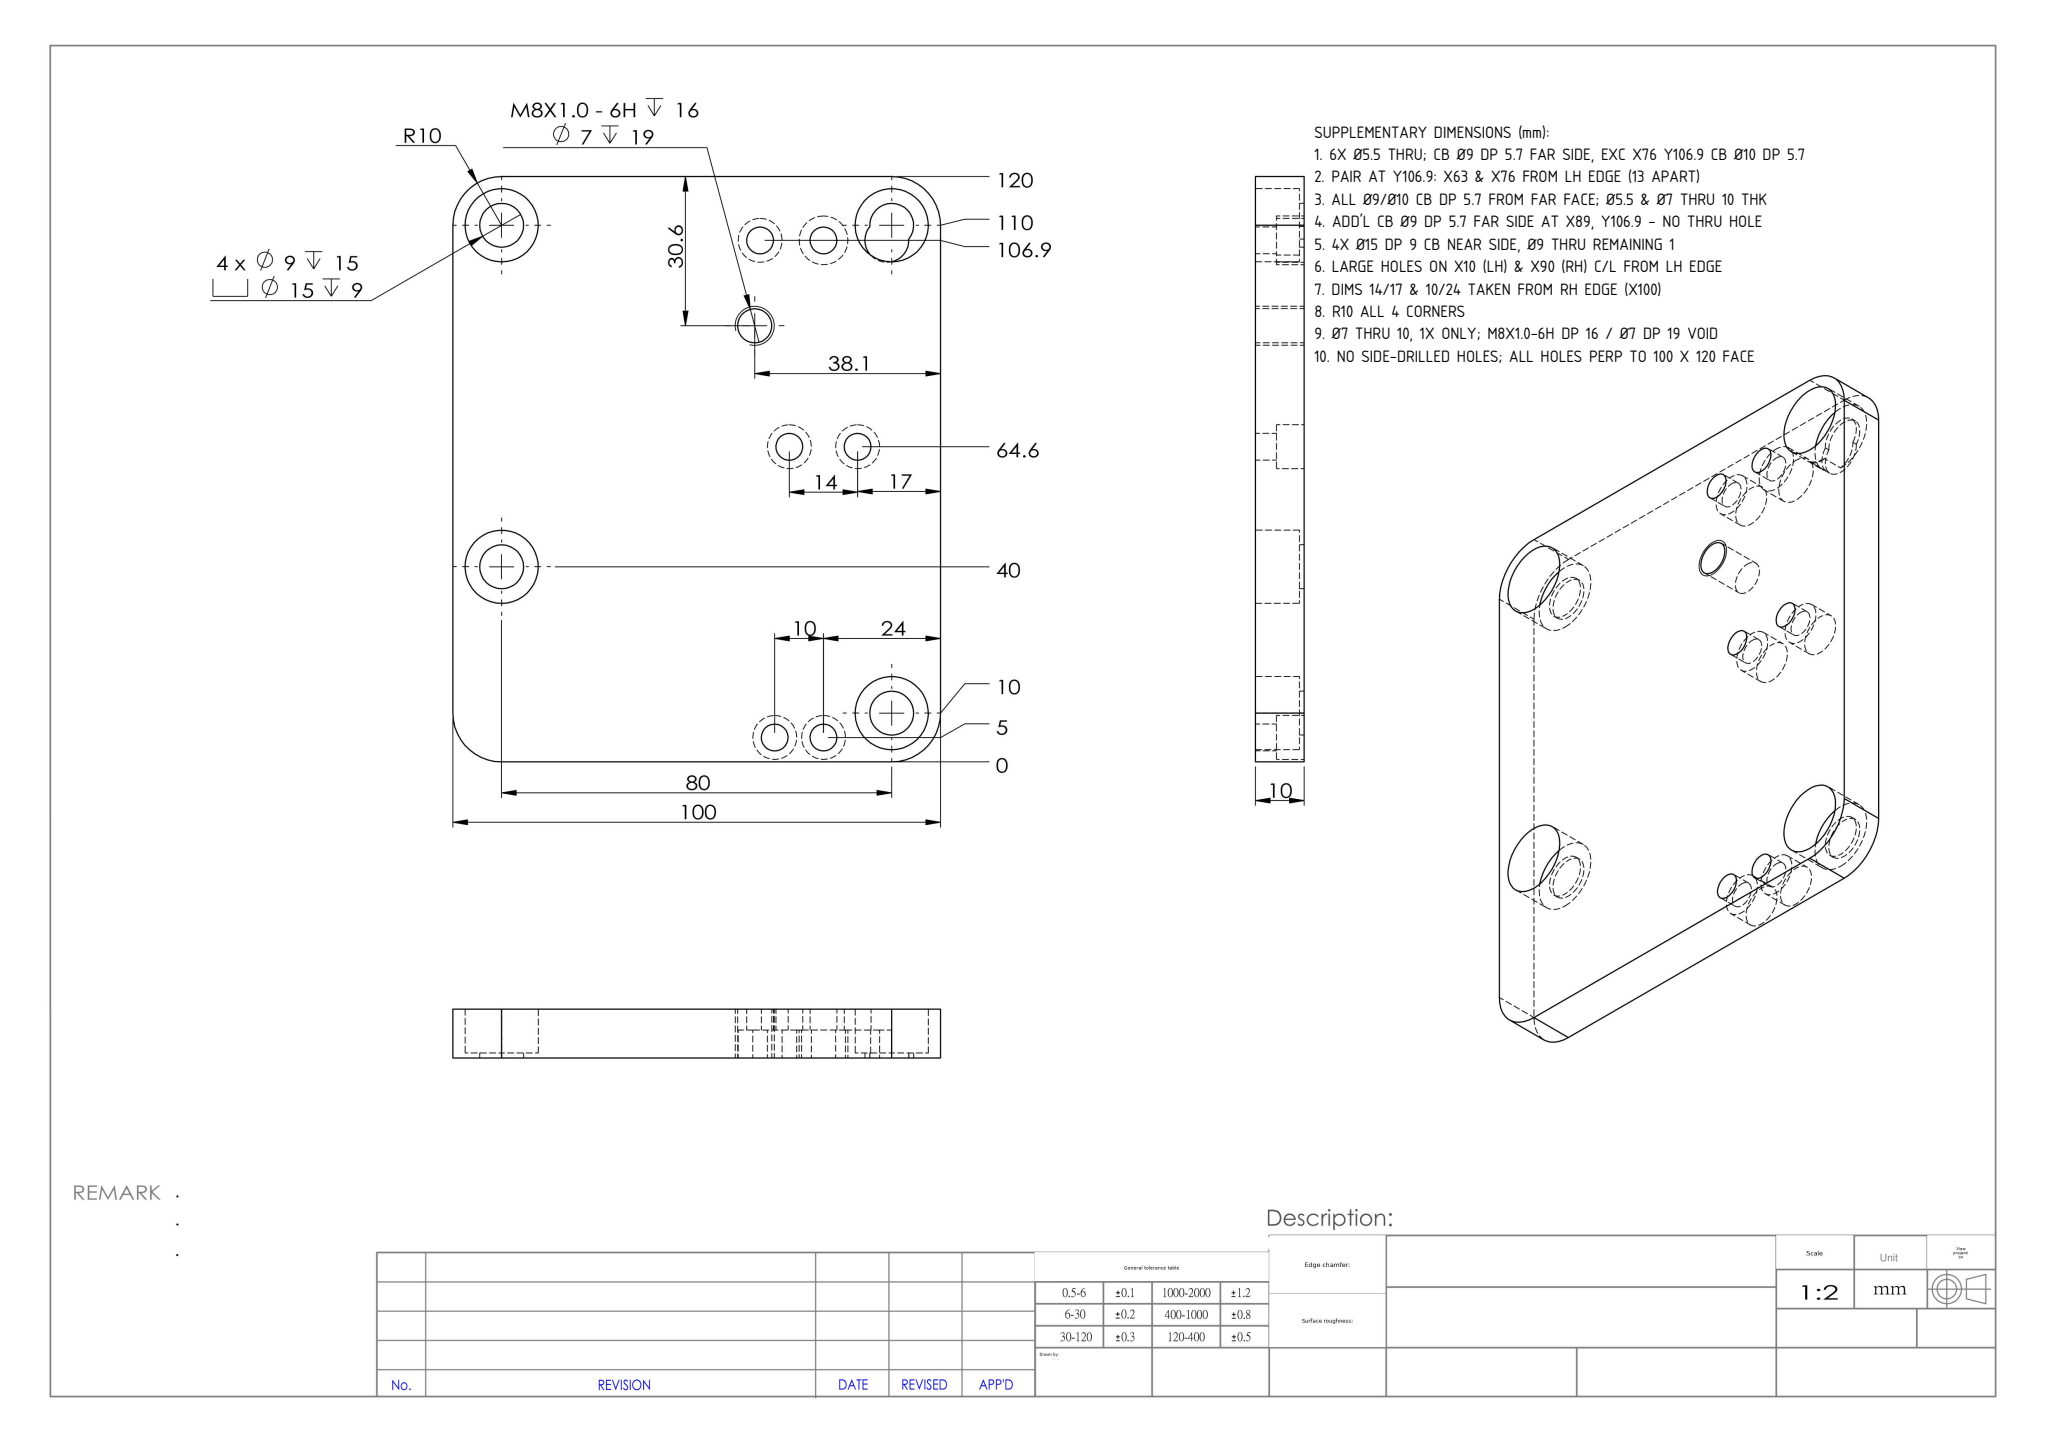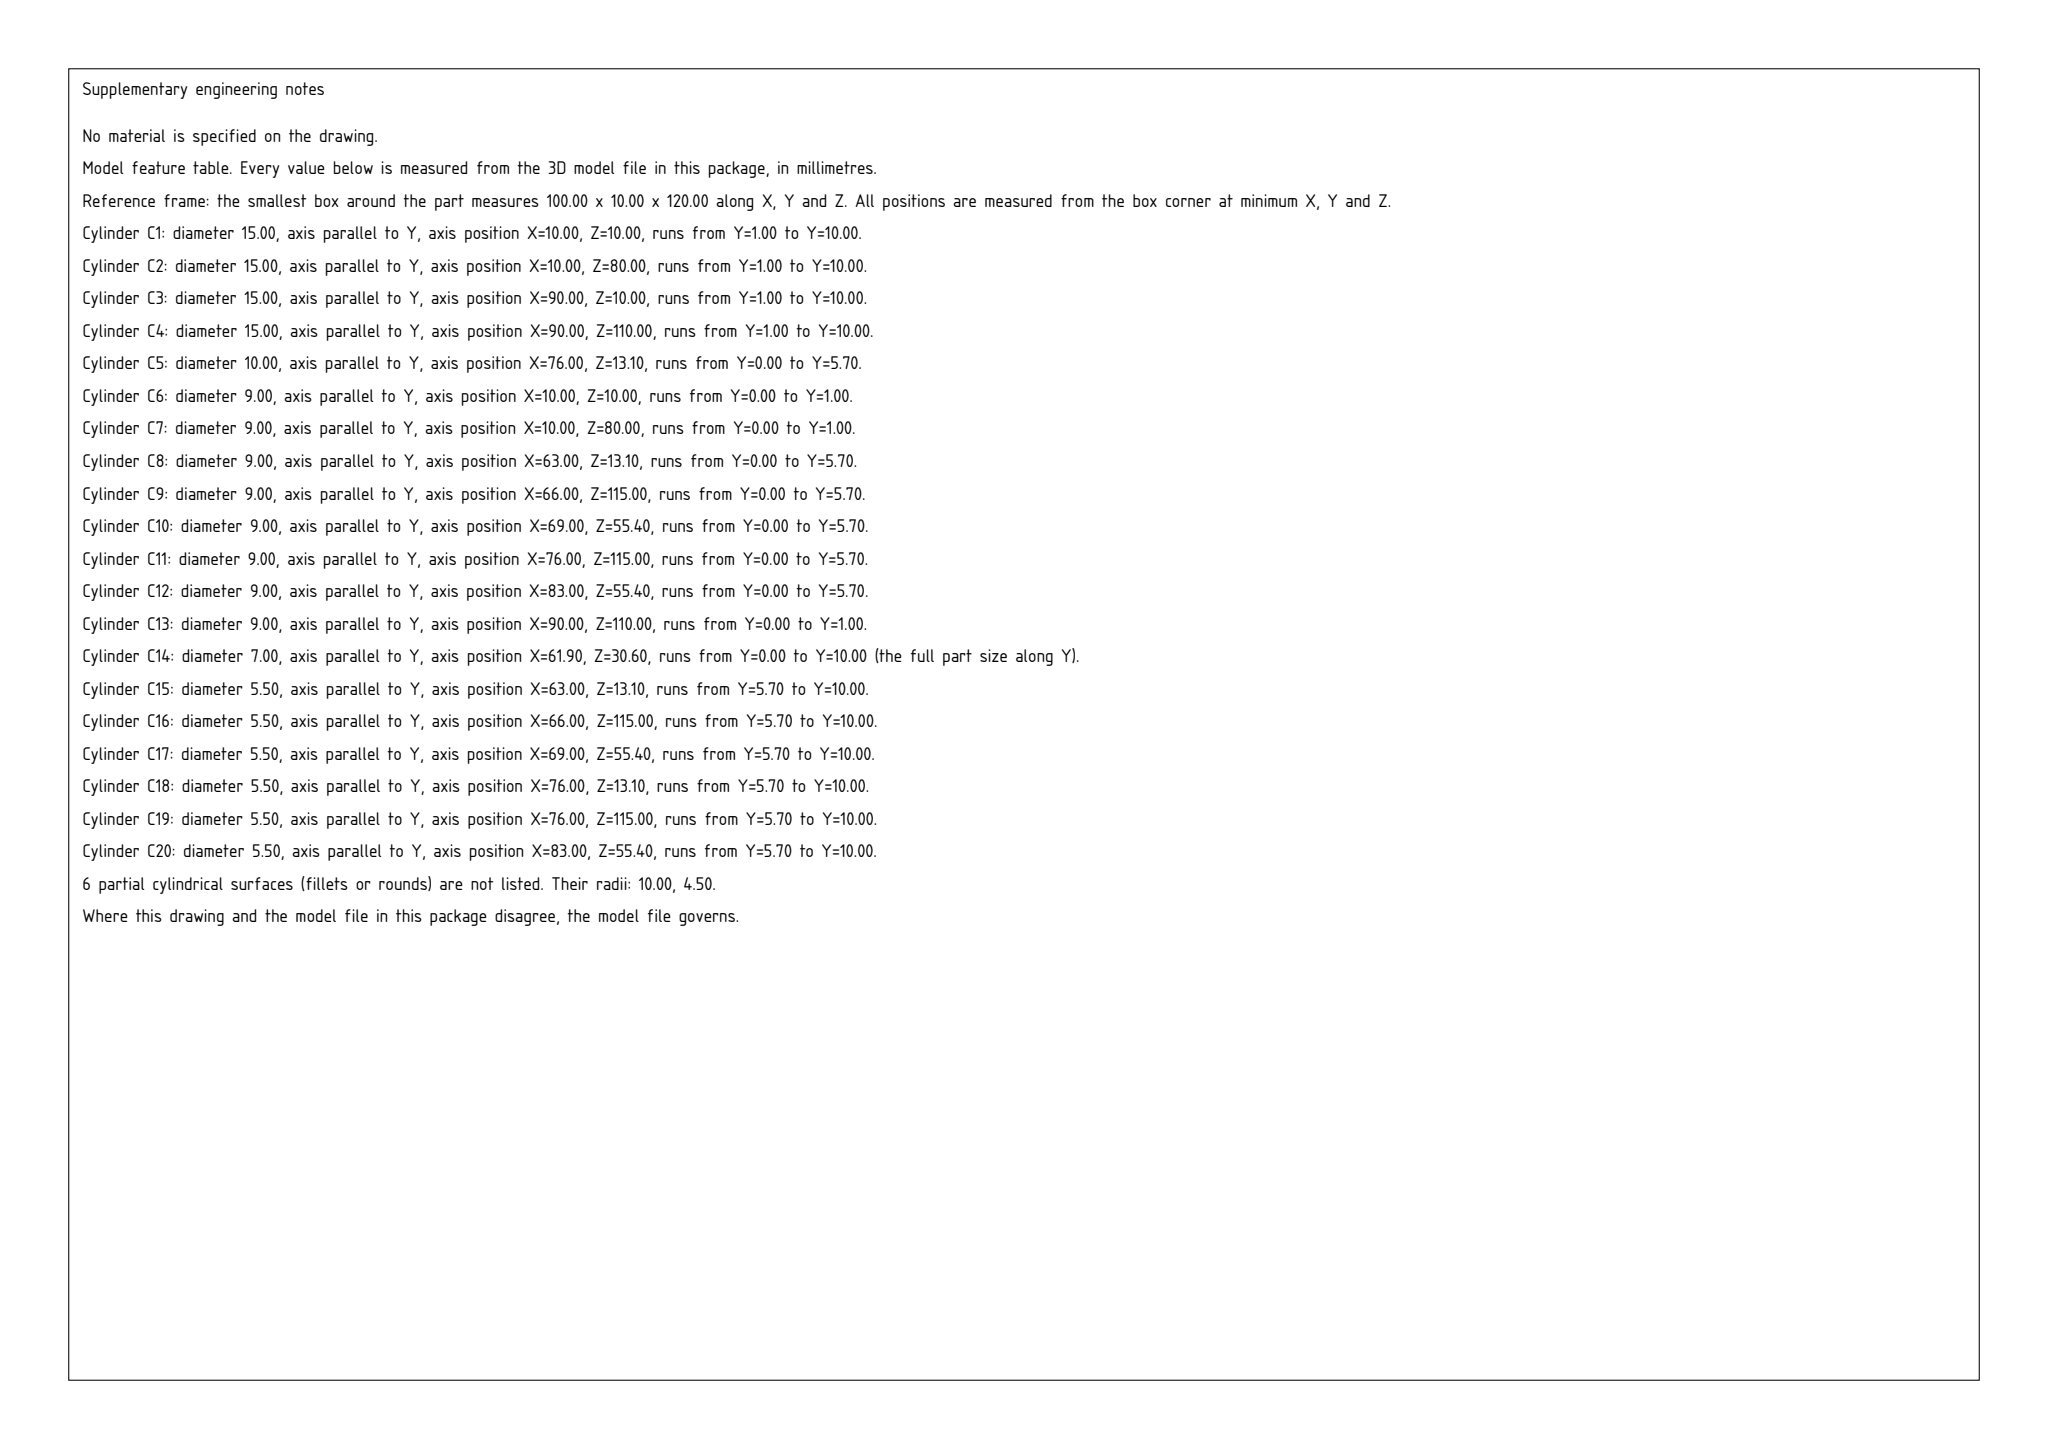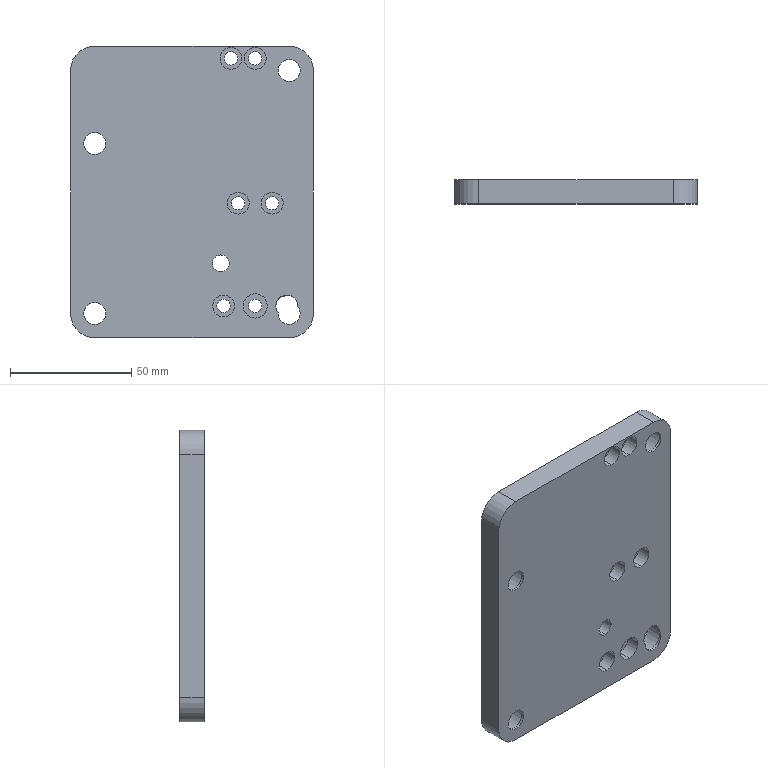Part | SolidWorks | mm | 1 solid | 63 faces | box 100 x 10 x 120 mm | volume 109234 mm3 | cylinder 46 | plane 17 | commonest cylinder face diameters 9 x18 5.5 x12 15 x8 20 x4 7 x2 10 x2
build123d program:
from build123d import *

# Parameters (mm, degrees)
SKETCH1_W                                         = 100
SKETCH1_H                                         = 120
BOSS_EXTRUDE1_DEPTH                               = 10
FILLET1_R                                         = 10
HOLE_SIZE_ACCORDING_TO_TYPE_2_HEX_SOC_D           = 9
HOLE_SIZE_ACCORDING_TO_TYPE_2_HEX_SOC_DEPTH       = 15
HOLE_SIZE_ACCORDING_TO_TYPE_2_HEX_SOC_CBORE_D     = 15
HOLE_SIZE_ACCORDING_TO_TYPE_2_HEX_SOC_CBORE_DEPTH = 9
HOLE_SIZE_ACCORDING_TO_TYPE_2_HEX_SOC_TIP         = 2.704
HOLE_SIZE_ACCORDING_TO_TYPE_7_HEX_SOC_D           = 5.5
HOLE_SIZE_ACCORDING_TO_TYPE_7_HEX_SOC_CBORE_D     = 9
HOLE_SIZE_ACCORDING_TO_TYPE_7_HEX_SOC_CBORE_DEPTH = 5.7
HOLE_SIZE_ACCORDING_TO_TYPE_8_HEX_SOC_D           = 5.5
HOLE_SIZE_ACCORDING_TO_TYPE_8_HEX_SOC_CBORE_D     = 10
HOLE_SIZE_ACCORDING_TO_TYPE_8_HEX_SOC_CBORE_DEPTH = 5.7
M8X1_0_TAPPED_HOLE1_D                             = 7
M8X1_0_TAPPED_HOLE1_DEPTH                         = 19
M8X1_0_TAPPED_HOLE1_TIP                           = 2.103


with BuildPart() as part:
    # Sketch1 → Boss-Extrude1 (new body)
    with BuildSketch(Plane(origin=(0, 0, 0), x_dir=(1, 0, 0), z_dir=(0, 1, 0))):
        Rectangle(SKETCH1_W, SKETCH1_H)
    extrude(amount=BOSS_EXTRUDE1_DEPTH)

    # Fillet1
    fillet1_edges = [part.edges().sort_by_distance(p)[0] for p in [
        (50, 5, 60),
        (-50, 5, 60),
        (-50, 5, -60),
        (50, 5, -60),
    ]]
    fillet(fillet1_edges, radius=FILLET1_R)

    # Hole Size _ according to_ Type 2 Hex Soc
    with Locations(Plane(origin=(0, 10, 0), x_dir=(1, 0, 0), z_dir=(0, 1, 0))):
        with Locations((-40, -20), (40, -50), (40, 50), (-40, 50)):
            CounterBoreHole(HOLE_SIZE_ACCORDING_TO_TYPE_2_HEX_SOC_D / 2, HOLE_SIZE_ACCORDING_TO_TYPE_2_HEX_SOC_CBORE_D / 2, HOLE_SIZE_ACCORDING_TO_TYPE_2_HEX_SOC_CBORE_DEPTH, depth=HOLE_SIZE_ACCORDING_TO_TYPE_2_HEX_SOC_DEPTH)
            with Locations((0, 0, -(HOLE_SIZE_ACCORDING_TO_TYPE_2_HEX_SOC_DEPTH + HOLE_SIZE_ACCORDING_TO_TYPE_2_HEX_SOC_TIP / 2))):  # 118° drill point
                Cone(0, HOLE_SIZE_ACCORDING_TO_TYPE_2_HEX_SOC_D / 2, HOLE_SIZE_ACCORDING_TO_TYPE_2_HEX_SOC_TIP, mode=Mode.SUBTRACT)

    # Hole Size _ according to_ Type 7 Hex Soc (through all)
    with Locations(Plane(origin=(0, 0, 0), x_dir=(-1, 0, 0), z_dir=(0, -1, 0))):
        with Locations((-26, -55), (-16, -55), (-19, 4.6), (-33, 4.6), (-13, 46.9), (-39, 46.9)):
            CounterBoreHole(HOLE_SIZE_ACCORDING_TO_TYPE_7_HEX_SOC_D / 2, HOLE_SIZE_ACCORDING_TO_TYPE_7_HEX_SOC_CBORE_D / 2, HOLE_SIZE_ACCORDING_TO_TYPE_7_HEX_SOC_CBORE_DEPTH)

    # Hole Size _ according to_ Type 8 Hex Soc (through all)
    with Locations(Plane(origin=(0, 0, 0), x_dir=(-1, 0, 0), z_dir=(0, -1, 0))):
        with Locations((-26, 46.9)):
            CounterBoreHole(HOLE_SIZE_ACCORDING_TO_TYPE_8_HEX_SOC_D / 2, HOLE_SIZE_ACCORDING_TO_TYPE_8_HEX_SOC_CBORE_D / 2, HOLE_SIZE_ACCORDING_TO_TYPE_8_HEX_SOC_CBORE_DEPTH)

    # M8x1.0 Tapped Hole1
    with Locations(Plane(origin=(0, 10, 0), x_dir=(1, 0, 0), z_dir=(0, 1, 0))):
        with Locations((11.9, 29.4)):
            Hole(M8X1_0_TAPPED_HOLE1_D / 2, depth=M8X1_0_TAPPED_HOLE1_DEPTH)
            with Locations((0, 0, -(M8X1_0_TAPPED_HOLE1_DEPTH + M8X1_0_TAPPED_HOLE1_TIP / 2))):  # 118° drill point
                Cone(0, M8X1_0_TAPPED_HOLE1_D / 2, M8X1_0_TAPPED_HOLE1_TIP, mode=Mode.SUBTRACT)


solid = part.part